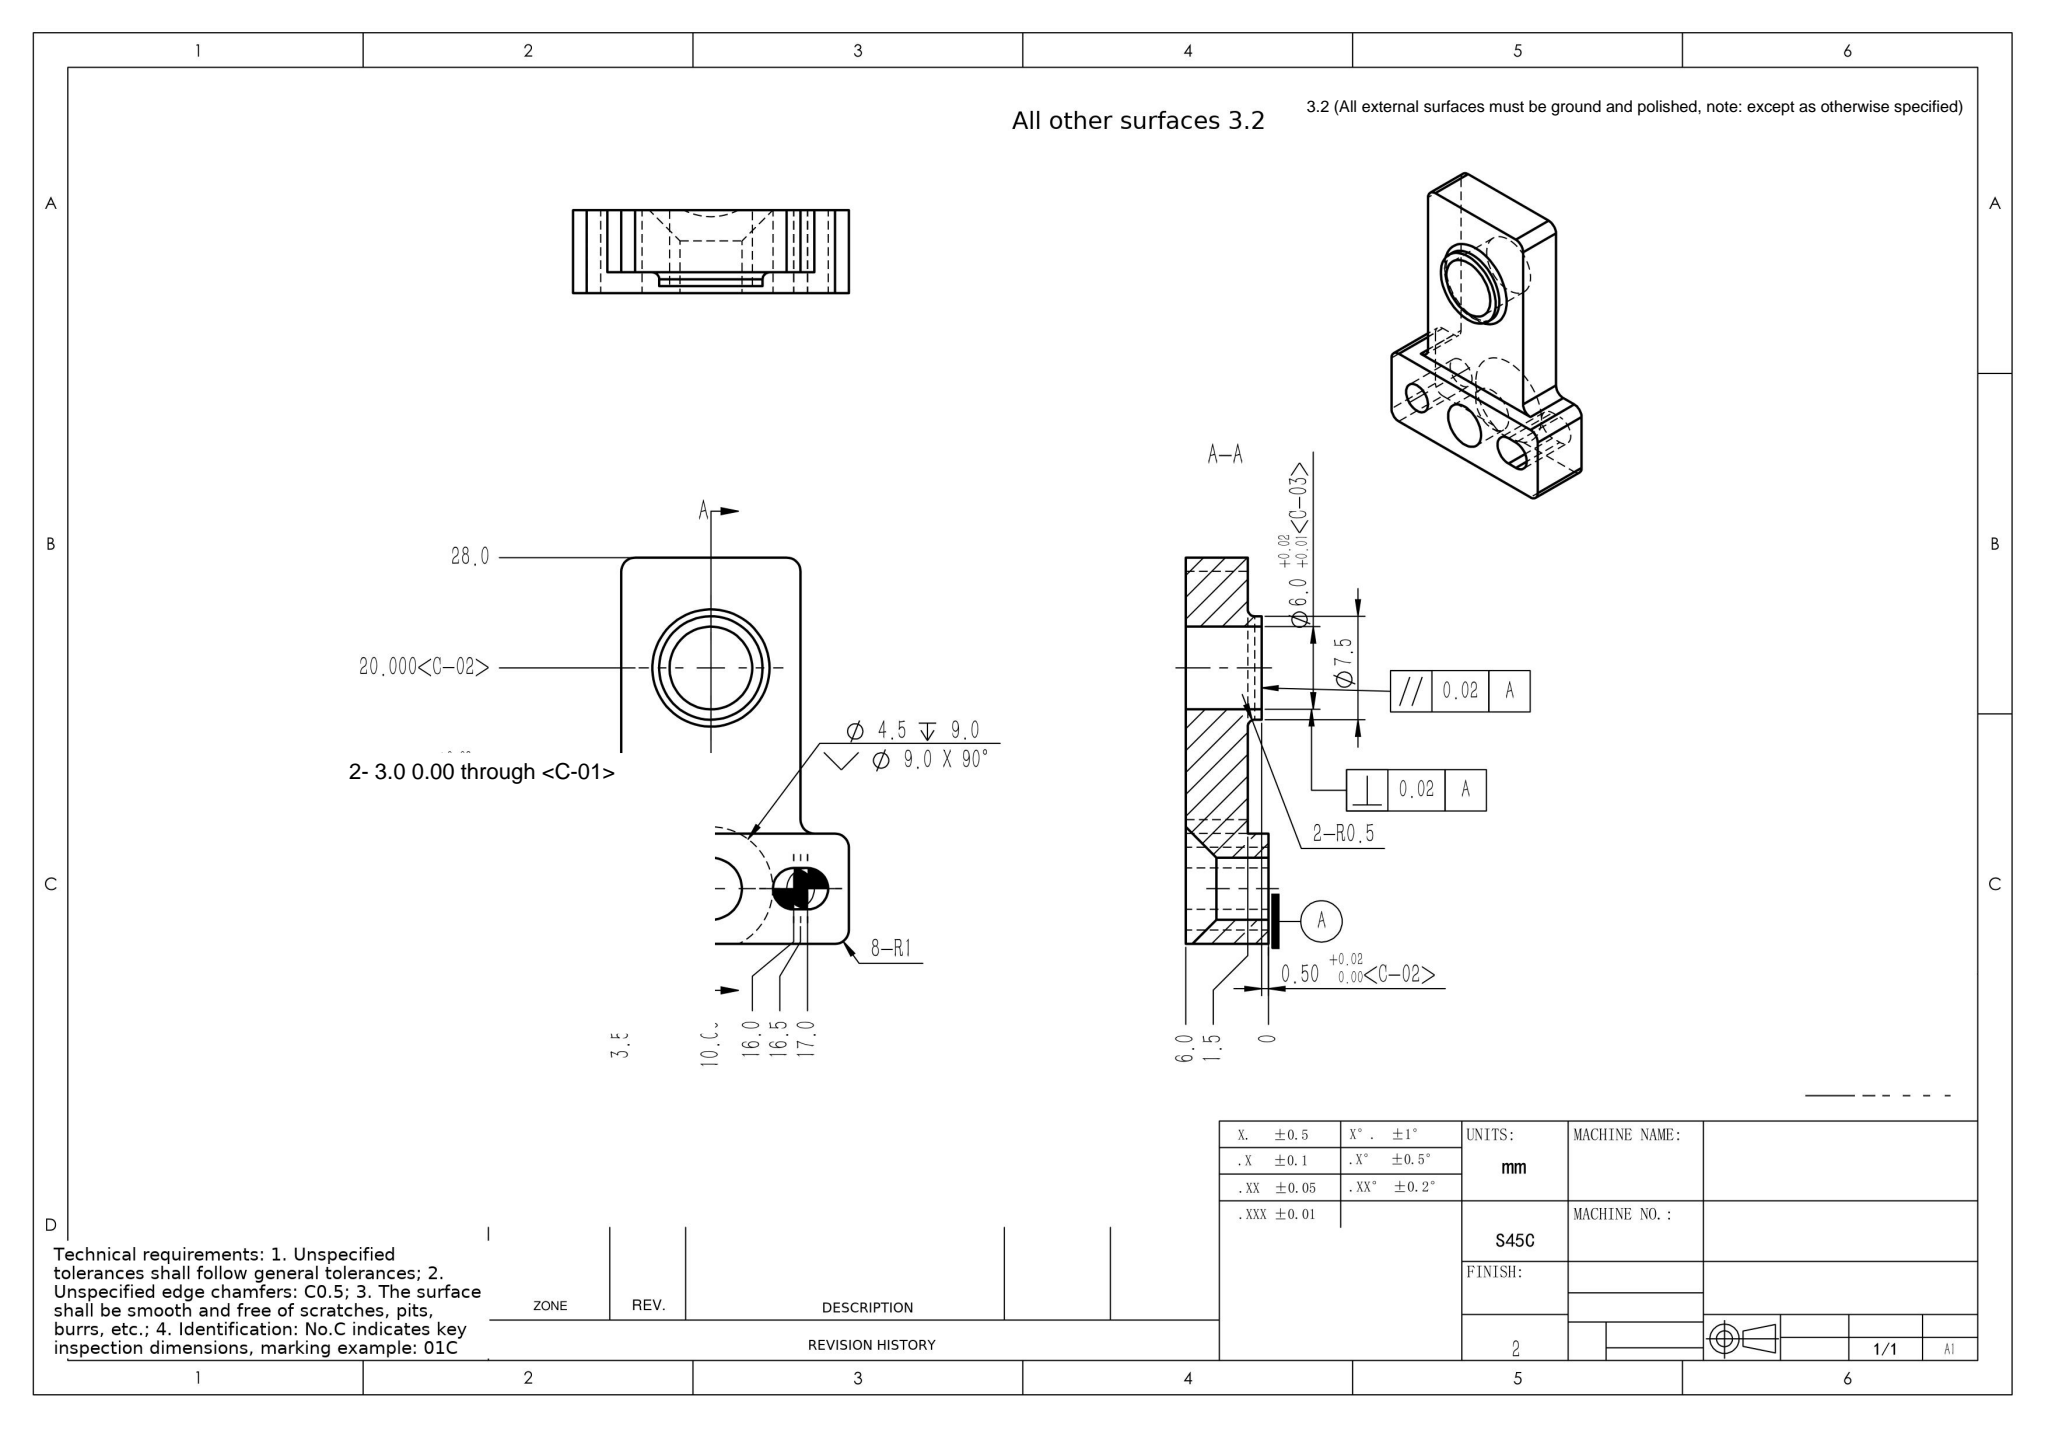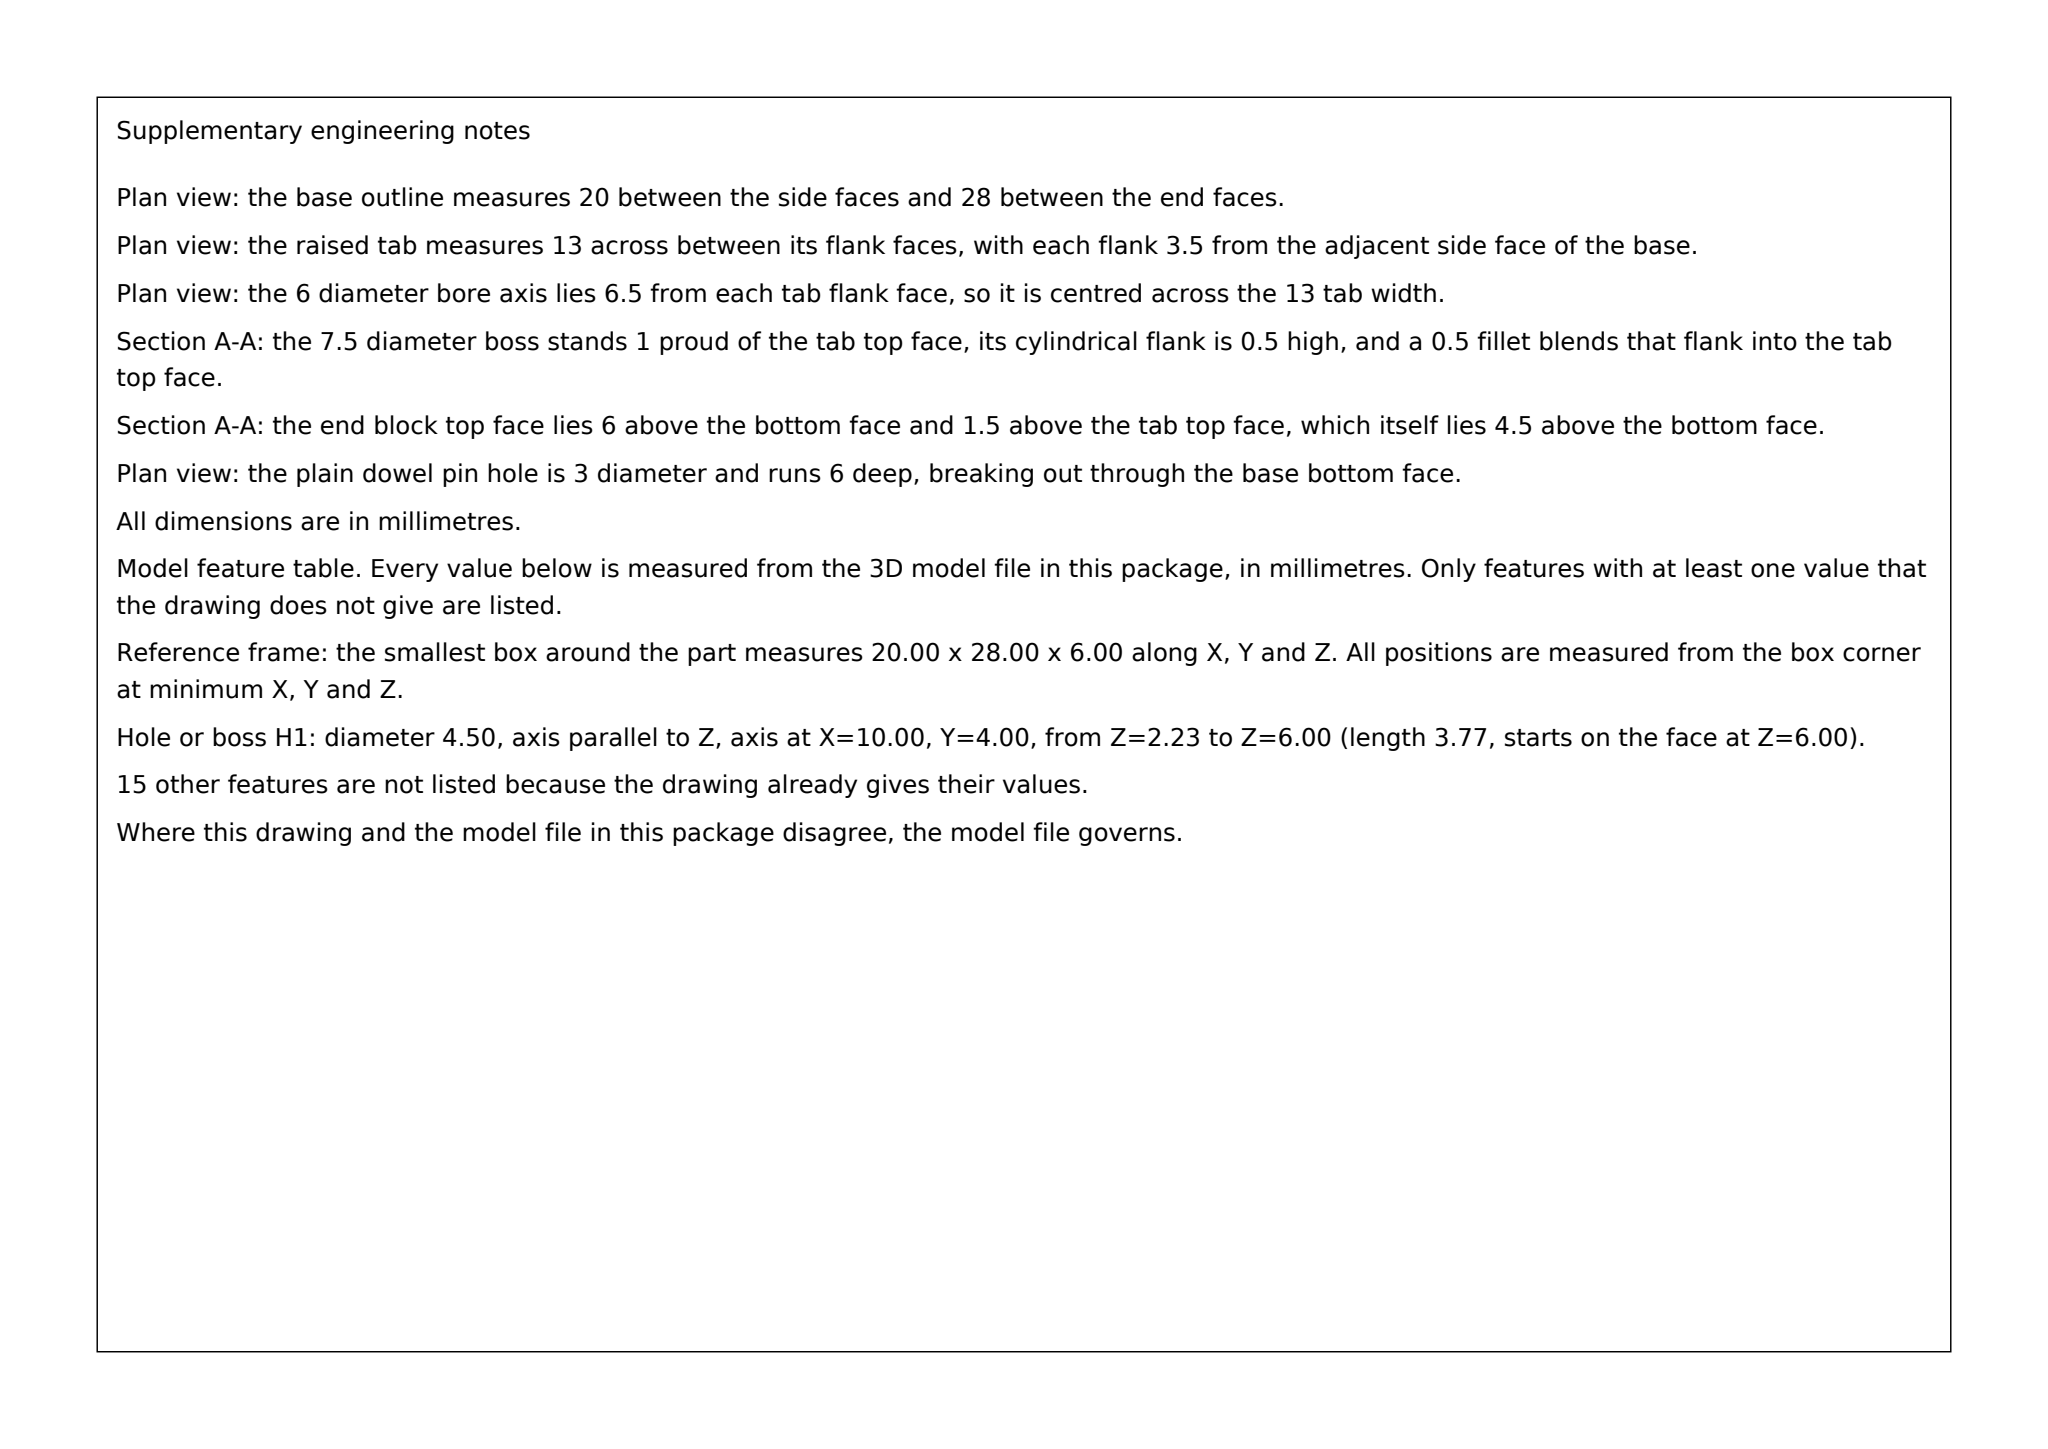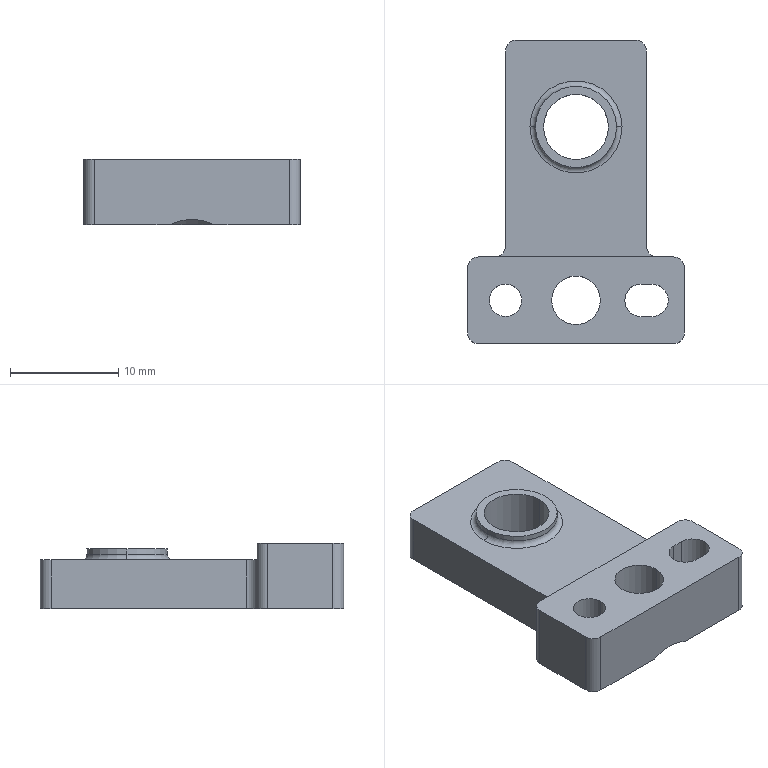Part | SolidWorks | mm | 1 solid | 36 faces | box 20 x 28 x 6 mm | volume 1770 mm3 | cylinder 19 | plane 13 | cone 2 | torus 2 | commonest cylinder face diameters 2 x8 3 x5 4.5 x2 7.5 x2 6 x2
Drawing notes:
Right base feature is an obround slot: 3.0 wide THRU 6.0, R1.5 end radii centered at X16.0 and X17.0, Y4.5 from base min-corner datum; overall slot length 4.0 | from the solid: cylinders: two 180-deg concave arcs dia 3.0, axis z at [16.0, 4.5] and [17.0, 4.5], from z0.0 to z6.0; axis_planes y=3.0 and y=6.0 each with extent x[16.0,17.0], z[0.0,6.0] (slot side walls, 3.0 wide, ends 14.5 to 18.5 = 4.0 long)
UPRIGHT PLATE THICKNESS 4.5 (Z0 to Z4.5); BASE THICKNESS 6.0 (Z0 to Z6.0) | from the solid: axis_planes: z=4.5 extent x[2.5,17.5] y[8.5,28.5]; x=3.5 and x=16.5 extents z[0.0,4.5]; z=6.0 extent x[0,20] y[0.5,8.5]
THICKNESS STEP 1.5 (Z4.5 TO Z6.0) LOCATED AT Y8.5 FROM BASE MIN-CORNER DATUM; 6.0 thick region Y0.5 to Y8.5, 4.5 thick region Y8.5 to Y28.5 | from the solid: axis_planes: y=8.5 extent x[1.0,19.0] z[0.0,6.0]; z=6.0 extent y[0.5,8.5]; z=4.5 extent y[8.5,28.5]
UPRIGHT PLATE FACE AT Z0 IS FLUSH WITH BASE BOTTOM FACE Z0; PLATE OPPOSITE FACE Z4.5 IS 1.5 BELOW BASE TOP FACE Z6.0 | from the solid: axis_planes: z=0.0 extent x[0,20] y[0.5,28.5] (common base+plate face); z=4.5 plate face; z=6.0 base top face
UPRIGHT PLATE WIDTH 13.0 (X3.5 TO X16.5 FROM BASE MIN-CORNER DATUM), 4.5 THK, EXTENDS TO Y28.5 | from the solid: axis_planes x=3.5 and x=16.5, each extent y[9.5,27.5] z[0,4.5]
BASE OVERALL WIDTH 20.0 (X0 TO X20.0 FROM BASE MIN-CORNER DATUM) | from the solid: bbox_xyz [20.0, 28.48, 6.0]; axis_planes x=0.0 and x=20.0, extent z[0,6.0]
1X Ø3.0 THRU (Z0 TO Z6.0), AXIS AT X3.5, Y4.5 FROM BASE MIN-CORNER DATUM | from the solid: cylinders hole/bore dia 3.0, axis z at [3.5, 4.5], from 0.0 to 6.0, 360 deg
UPRIGHT PLATE WIDTH 13.0 (X3.5 TO X16.5 FROM BASE MIN-CORNER DATUM), CENTERED AT X10.0; PLATE HEIGHT TO Y28.5, THICKNESS 4.5 (Z0 TO Z4.5) | from the solid: axis_planes x=3.5 and x=16.5, extent y[9.5,27.5] z[0,4.5]
BASE OVERALL WIDTH 20.0 (X0 TO X20.0), DEPTH Y0.5 TO Y8.5, THICKNESS 6.0 (Z0 TO Z6.0) | from the solid: axis_planes z=0 extent x[0,20] y[0.5,28.5]; z=6.0 extent x[0,20] y[0.5,8.5]
Ø3.0 THRU (Z0 TO Z6.0), HOLE AXIS AT X3.5, Y4.5 FROM BASE MIN-CORNER DATUM | from the solid: cylinders hole/bore dia 3.0 axis z at [3.5,4.5], from 0.0 to 6.0
OPPOSITE END FEATURE: 3.0 WIDE OBROUND SLOT THRU (Z0 TO Z6.0), R1.5 ENDS AT X16.0 AND X17.0, Y4.5 FROM BASE MIN-CORNER DATUM | from the solid: cylinders concave arc dia 3.0 axis z at [16.0,4.5] and [17.0,4.5], from 0.0 to 6.0, arc 180
build123d program:
from build123d import *

# Parameters (mm, degrees)
SKETCH1_W                                            = 20
SKETCH1_H                                            = 28
BOSS_EXTRUDE1_DEPTH                                  = 4.5
SIZE_MM_DOWEL_PIN_HOLE1_D                            = 3
SIZE_MM_DOWEL_PIN_HOLE1_DEPTH                        = 6
SKETCH3_R                                            = 3
CUT_EXTRUDE4_DEPTH                                   = 4.5
BOSS_EXTRUDE2_START                                  = 1
SKETCH9_R                                            = 3.75
SKETCH9_R_2                                          = 3
BOSS_EXTRUDE2_DEPTH                                  = 1
FILLET2_R                                            = 0.5
BOSS_EXTRUDE3_START                                  = 1.5
SKETCH10_W                                           = 20
SKETCH10_H                                           = 8
SKETCH10_R                                           = 1.5
BOSS_EXTRUDE3_DEPTH                                  = 1.5
CUT_EXTRUDE5_DEPTH                                   = 4.5
FILLET3_R                                            = 1
CUT_EXTRUDE6_DEPTH                                   = 6
SKETCH14_R                                           = 2.25
CUT_EXTRUDE7_DEPTH                                   = 6
M4_HEXAGONAL_COUNTERSUNK_SCREW_COUNTERSU_D           = 4.5
M4_HEXAGONAL_COUNTERSUNK_SCREW_COUNTERSU_DEPTH       = 9
M4_HEXAGONAL_COUNTERSUNK_SCREW_COUNTERSU_CSINK_D     = 8.96
M4_HEXAGONAL_COUNTERSUNK_SCREW_COUNTERSU_CSINK_ANGLE = 90
M4_HEXAGONAL_COUNTERSUNK_SCREW_COUNTERSU_TIP         = 1.352


with BuildPart() as part:
    # Sketch1 → Boss-Extrude1 (new body)
    with BuildSketch(Plane.XY):
        Rectangle(SKETCH1_W, SKETCH1_H)
    extrude(amount=BOSS_EXTRUDE1_DEPTH)

    # Size mm Dowel Pin Hole1
    with Locations(Plane(origin=(0, 0, 0), x_dir=(-1, 0, 0), z_dir=(0, 0, -1))):
        with Locations((-6.5, -10), (6.5, -10)):
            Hole(SIZE_MM_DOWEL_PIN_HOLE1_D / 2, depth=SIZE_MM_DOWEL_PIN_HOLE1_DEPTH)

    # Sketch3 → Cut-Extrude4 (cut)
    with BuildSketch(Plane.XY.offset(4.5)):
        with Locations((0, 6)):
            Circle(SKETCH3_R)
    extrude(amount=-CUT_EXTRUDE4_DEPTH, mode=Mode.SUBTRACT)

    # Sketch9 → Boss-Extrude2 (add)
    with BuildSketch(Plane.XY.offset(4.5).offset(BOSS_EXTRUDE2_START)):
        with Locations((0, 6)):
            Circle(SKETCH9_R)
        with Locations((0, 6)):
            Circle(SKETCH9_R_2, mode=Mode.SUBTRACT)
    extrude(amount=-BOSS_EXTRUDE2_DEPTH)

    # Fillet2
    fillet2_edges = [part.edges().sort_by_distance(p)[0] for p in [
        (-3.75, 6, 4.5),
    ]]
    fillet(fillet2_edges, radius=FILLET2_R)

    # Sketch10 → Boss-Extrude3 (add)
    with BuildSketch(Plane.XY.offset(4.5).offset(BOSS_EXTRUDE3_START)):
        with Locations((0, -10)):
            Rectangle(SKETCH10_W, SKETCH10_H)
        with Locations(Location((-6.5, -10, 0), (0, 0, 180))):
            Circle(SKETCH10_R, mode=Mode.SUBTRACT)
        with Locations(Location((6.5, -10, 0), (0, 0, 180))):
            Circle(SKETCH10_R, mode=Mode.SUBTRACT)
    extrude(amount=-BOSS_EXTRUDE3_DEPTH)

    # Sketch11 → Cut-Extrude5 (cut)
    with BuildSketch(Plane.XY.offset(4.5)):
        with BuildLine():
            Line((-10, 14), (-6.5, 14))
            Line((-6.5, 14), (-6.5, -5))
            ThreePointArc((-6.5, -5), (-6.793, -5.707), (-7.5, -6))
            Line((-7.5, -6), (-10, -6))
            Line((-10, -6), (-10, 14))
        make_face()
        with BuildLine():
            Line((10, 14), (6.5, 14))
            Line((6.5, 14), (6.5, -5))
            ThreePointArc((6.5, -5), (6.793, -5.707), (7.5, -6))
            Line((7.5, -6), (10, -6))
            Line((10, -6), (10, 14))
        make_face()
    extrude(amount=-CUT_EXTRUDE5_DEPTH, mode=Mode.SUBTRACT)

    # Fillet3
    fillet3_edges = [part.edges().sort_by_distance(p)[0] for p in [
        (-10, -6, 3),
        (10, -6, 3),
        (-6.5, 14, 2.25),
        (10, -14, 3),
        (-10, -14, 3),
        (6.5, 14, 2.25),
    ]]
    fillet(fillet3_edges, radius=FILLET3_R)

    # Sketch12 → Cut-Extrude6 (cut)
    with BuildSketch(Plane(origin=(0, 0, 0), x_dir=(-1, 0, 0), z_dir=(0, 0, -1))):
        with BuildLine():
            Line((-7, -8.5), (-6, -8.5))
            ThreePointArc((-6, -8.5), (-4.5, -10), (-6, -11.5))
            Line((-6, -11.5), (-7, -11.5))
            ThreePointArc((-7, -11.5), (-8.5, -10), (-7, -8.5))
        make_face()
    extrude(amount=-CUT_EXTRUDE6_DEPTH, mode=Mode.SUBTRACT)

    # Sketch14 → Cut-Extrude7 (cut)
    with BuildSketch(Plane(origin=(0, 0, 0), x_dir=(-1, 0, 0), z_dir=(0, 0, -1))):
        with Locations((0, -10)):
            Circle(SKETCH14_R)
    extrude(amount=-CUT_EXTRUDE7_DEPTH, mode=Mode.SUBTRACT)

    # M4 Hexagonal Countersunk Screw Countersu
    with Locations(Plane(origin=(0, -10, 0), x_dir=(-1, 0, 0), z_dir=(0, 0, -1))):
        with Locations((0, 0)):
            CounterSinkHole(M4_HEXAGONAL_COUNTERSUNK_SCREW_COUNTERSU_D / 2, M4_HEXAGONAL_COUNTERSUNK_SCREW_COUNTERSU_CSINK_D / 2, depth=M4_HEXAGONAL_COUNTERSUNK_SCREW_COUNTERSU_DEPTH, counter_sink_angle=M4_HEXAGONAL_COUNTERSUNK_SCREW_COUNTERSU_CSINK_ANGLE)
            with Locations((0, 0, -(M4_HEXAGONAL_COUNTERSUNK_SCREW_COUNTERSU_DEPTH + M4_HEXAGONAL_COUNTERSUNK_SCREW_COUNTERSU_TIP / 2))):  # 118° drill point
                Cone(0, M4_HEXAGONAL_COUNTERSUNK_SCREW_COUNTERSU_D / 2, M4_HEXAGONAL_COUNTERSUNK_SCREW_COUNTERSU_TIP, mode=Mode.SUBTRACT)


solid = part.part